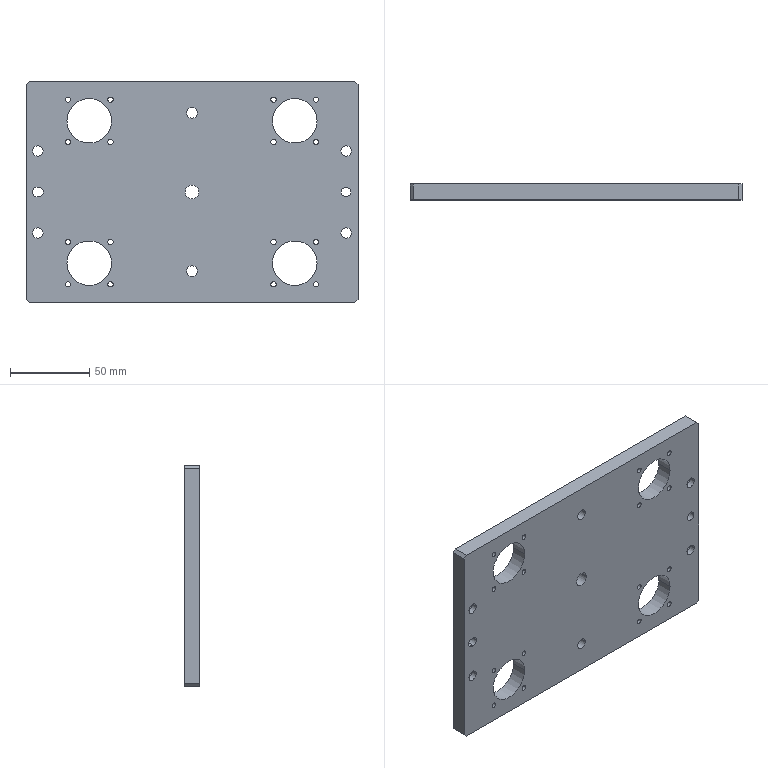Component | SolidWorks | 20-MaterialTrayLifting-1111-1_21-1111-1 | 1 solid | 83 faces | box 210 x 10 x 140 mm | volume 262683 mm3 | cylinder 67 | plane 16 | commonest cylinder face diameters 3.3 x32 11 x8 6.6 x8 28.2 x8 6 x5 6.8 x4 8.8 x2 | material S45C
build123d program:
from build123d import *

# Parameters (mm, degrees)
SKETCH1_W                                       = 210
SKETCH1_H                                       = 140
BOSS_EXTRUDE1_DEPTH                             = 10
SKETCH2_R                                       = 14.1
CUT_EXTRUDE1_DEPTH                              = 127.59
SKETCH5_R                                       = 3
CUT_EXTRUDE2_DEPTH                              = 127.59
M6_HEX_SOCKET_HEAD_CAP_SCREW_CBORE1_D           = 6.6
M6_HEX_SOCKET_HEAD_CAP_SCREW_CBORE1_CBORE_D     = 11
M6_HEX_SOCKET_HEAD_CAP_SCREW_CBORE1_CBORE_DEPTH = 6.4
SIZE_MM_DOWEL_PIN_HOLE_1_D                      = 6
CHAMFER1_SIZE                                   = 2
CUT_EXTRUDE4_DEPTH                              = 127.59
M8_TAPPED_HOLE1_D                               = 6.8
M4_TAPPED_HOLE1_AT_2_COUNT                      = 2
M4_TAPPED_HOLE1_AT_2_PITCH                      = 26.87
M4_TAPPED_HOLE1_AT_3_COUNT                      = 2
M4_TAPPED_HOLE1_AT_3_PITCH                      = 38
M4_TAPPED_HOLE1_AT_4_COUNT                      = 2
M4_TAPPED_HOLE1_AT_4_PITCH                      = 26.87
M10X1_25_TAPPED_HOLE1_D                         = 8.8


with BuildPart() as part:
    # Sketch1 → Boss-Extrude1 (new body)
    with BuildSketch(Plane.XY):
        Rectangle(SKETCH1_W, SKETCH1_H)
    extrude(amount=BOSS_EXTRUDE1_DEPTH)

    # Sketch2 → Cut-Extrude1 (cut, through all)
    with BuildSketch(Plane.XY.offset(10)):
        with Locations((-65, 45)):
            Circle(SKETCH2_R)
        with Locations((65, 45)):
            Circle(SKETCH2_R)
        with Locations((-65, -45)):
            Circle(SKETCH2_R)
        with Locations((65, -45)):
            Circle(SKETCH2_R)
    extrude(amount=-CUT_EXTRUDE1_DEPTH, mode=Mode.SUBTRACT)

    # Sketch5 → Cut-Extrude2 (cut, through all)
    with BuildSketch(Plane.XY.offset(10)):
        Circle(SKETCH5_R)
    extrude(amount=-CUT_EXTRUDE2_DEPTH, mode=Mode.SUBTRACT)

    # M6 Hex Socket Head Cap Screw CBORE1 (through all)
    with Locations(Plane.XY.offset(10)):
        with Locations((-97.5, 78), (-97.5, 26), (-97.5, -26), (-97.5, -78), (97.5, 78), (97.5, 26), (97.5, -26), (97.5, -78)):
            CounterBoreHole(M6_HEX_SOCKET_HEAD_CAP_SCREW_CBORE1_D / 2, M6_HEX_SOCKET_HEAD_CAP_SCREW_CBORE1_CBORE_D / 2, M6_HEX_SOCKET_HEAD_CAP_SCREW_CBORE1_CBORE_DEPTH)

    # Size mm Dowel Pin Hole 1 (through all)
    with Locations(Plane.XY.offset(10)):
        with Locations((-97.5, 0), (97.5, 0)):
            Hole(SIZE_MM_DOWEL_PIN_HOLE_1_D / 2)

    # Chamfer1
    chamfer1_edges = [part.edges().sort_by_distance(p)[0] for p in [
        (105, -70, 5),
        (-105, -70, 5),
        (-105, 70, 5),
        (105, 70, 5),
    ]]
    chamfer(chamfer1_edges, length=CHAMFER1_SIZE)

    # Sketch17 → Cut-Extrude4 (cut, through all)
    with BuildSketch(Plane.XY.offset(10)):
        with BuildLine():
            Line((-98, 3), (-97, 3))
            ThreePointArc((-97, 3), (-94, 0), (-97, -3))
            Line((-97, -3), (-98, -3))
            ThreePointArc((-98, -3), (-101, 0), (-98, 3))
        make_face()
    extrude(amount=-CUT_EXTRUDE4_DEPTH, mode=Mode.SUBTRACT)

    # M8 Tapped Hole1 (through all)
    with Locations(Plane.XY.offset(10)):
        with Locations((0, -50), (0, 50)):
            Hole(M8_TAPPED_HOLE1_D / 2)

    # Sketch23 → M4 Tapped Hole1 (revolve, cut)
    with BuildSketch(Plane(origin=(-78.435, -31.565, 10), x_dir=(0, -1, 0), z_dir=(1, 0, 0))):
        Polygon((0, 0), (0, 11.091), (1.65, 10.1), (1.65, 0), align=None)
    m4_tapped_hole1 = revolve(axis=Axis((-78.435, -31.565, 16.35), (0, 0, -1)), mode=Mode.SUBTRACT)

    # M4 Tapped Hole1 at 2: M4 Tapped Hole1 ×2
    with Locations(*[(0, -i * M4_TAPPED_HOLE1_AT_2_PITCH, 0) for i in range(1, M4_TAPPED_HOLE1_AT_2_COUNT)]):
        add(m4_tapped_hole1, mode=Mode.SUBTRACT)

    # M4 Tapped Hole1 at 3: M4 Tapped Hole1 ×2
    with Locations(*[Vector(0.7071, -0.7071, 0) * (i * M4_TAPPED_HOLE1_AT_3_PITCH) for i in range(1, M4_TAPPED_HOLE1_AT_3_COUNT)]):
        add(m4_tapped_hole1, mode=Mode.SUBTRACT)

    # M4 Tapped Hole1 at 4: M4 Tapped Hole1 ×2
    with Locations(*[(i * M4_TAPPED_HOLE1_AT_4_PITCH, 0, 0) for i in range(1, M4_TAPPED_HOLE1_AT_4_COUNT)]):
        add(m4_tapped_hole1, mode=Mode.SUBTRACT)

    # Mirror1: M4 Tapped Hole1 across plane
    add(m4_tapped_hole1.mirror(Plane.ZX), mode=Mode.SUBTRACT)

    # Mirror1 copy 1 sketch → Mirror1 copy 1 (revolve, cut)
    with BuildSketch(Plane(origin=(-78.435, 58.435, 10), x_dir=(0, 1, 0), z_dir=(1, 0, 0))):
        Polygon((0, 0), (0, -11.091), (1.65, -10.1), (1.65, 0), align=None)
    revolve(axis=Axis((-78.435, 58.435, 16.35), (0, 0, 1)), mode=Mode.SUBTRACT)

    # Mirror1 copy 2 sketch → Mirror1 copy 2 (revolve, cut)
    with BuildSketch(Plane(origin=(-51.565, 58.435, 10), x_dir=(0, 1, 0), z_dir=(1, 0, 0))):
        Polygon((0, 0), (0, -11.091), (1.65, -10.1), (1.65, 0), align=None)
    revolve(axis=Axis((-51.565, 58.435, 16.35), (0, 0, 1)), mode=Mode.SUBTRACT)

    # Mirror1 copy 3 sketch → Mirror1 copy 3 (revolve, cut)
    with BuildSketch(Plane(origin=(-51.565, 31.565, 10), x_dir=(0, 1, 0), z_dir=(1, 0, 0))):
        Polygon((0, 0), (0, -11.091), (1.65, -10.1), (1.65, 0), align=None)
    revolve(axis=Axis((-51.565, 31.565, 16.35), (0, 0, 1)), mode=Mode.SUBTRACT)

    # Mirror2: M4 Tapped Hole1 across plane
    add(m4_tapped_hole1.mirror(Plane(origin=(0, 0, 0), x_dir=(0, 0, 1), z_dir=(1, 0, 0))), mode=Mode.SUBTRACT)

    # Mirror2 copy 1 sketch → Mirror2 copy 1 (revolve, cut)
    with BuildSketch(Plane(origin=(78.435, -58.435, 10), x_dir=(0, -1, 0), z_dir=(-1, 0, 0))):
        Polygon((0, 0), (0, -11.091), (1.65, -10.1), (1.65, 0), align=None)
    revolve(axis=Axis((78.435, -58.435, 16.35), (0, 0, 1)), mode=Mode.SUBTRACT)

    # Mirror2 copy 2 sketch → Mirror2 copy 2 (revolve, cut)
    with BuildSketch(Plane(origin=(51.565, -58.435, 10), x_dir=(0, -1, 0), z_dir=(-1, 0, 0))):
        Polygon((0, 0), (0, -11.091), (1.65, -10.1), (1.65, 0), align=None)
    revolve(axis=Axis((51.565, -58.435, 16.35), (0, 0, 1)), mode=Mode.SUBTRACT)

    # Mirror2 copy 3 sketch → Mirror2 copy 3 (revolve, cut)
    with BuildSketch(Plane(origin=(51.565, -31.565, 10), x_dir=(0, -1, 0), z_dir=(-1, 0, 0))):
        Polygon((0, 0), (0, -11.091), (1.65, -10.1), (1.65, 0), align=None)
    revolve(axis=Axis((51.565, -31.565, 16.35), (0, 0, 1)), mode=Mode.SUBTRACT)

    # Mirror2 copy 4 sketch → Mirror2 copy 4 (revolve, cut)
    with BuildSketch(Plane(origin=(78.435, 31.565, 10), x_dir=(0, 1, 0), z_dir=(-1, 0, 0))):
        Polygon((0, 0), (0, 11.091), (1.65, 10.1), (1.65, 0), align=None)
    revolve(axis=Axis((78.435, 31.565, 16.35), (0, 0, -1)), mode=Mode.SUBTRACT)

    # Mirror2 copy 5 sketch → Mirror2 copy 5 (revolve, cut)
    with BuildSketch(Plane(origin=(78.435, 58.435, 10), x_dir=(0, 1, 0), z_dir=(-1, 0, 0))):
        Polygon((0, 0), (0, 11.091), (1.65, 10.1), (1.65, 0), align=None)
    revolve(axis=Axis((78.435, 58.435, 16.35), (0, 0, -1)), mode=Mode.SUBTRACT)

    # Mirror2 copy 6 sketch → Mirror2 copy 6 (revolve, cut)
    with BuildSketch(Plane(origin=(51.565, 58.435, 10), x_dir=(0, 1, 0), z_dir=(-1, 0, 0))):
        Polygon((0, 0), (0, 11.091), (1.65, 10.1), (1.65, 0), align=None)
    revolve(axis=Axis((51.565, 58.435, 16.35), (0, 0, -1)), mode=Mode.SUBTRACT)

    # Mirror2 copy 7 sketch → Mirror2 copy 7 (revolve, cut)
    with BuildSketch(Plane(origin=(51.565, 31.565, 10), x_dir=(0, 1, 0), z_dir=(-1, 0, 0))):
        Polygon((0, 0), (0, 11.091), (1.65, 10.1), (1.65, 0), align=None)
    revolve(axis=Axis((51.565, 31.565, 16.35), (0, 0, -1)), mode=Mode.SUBTRACT)

    # M10x1.25 Tapped Hole1 (through all)
    with Locations(Plane.XY.offset(10)):
        with Locations((0, 0)):
            Hole(M10X1_25_TAPPED_HOLE1_D / 2)


solid = part.part

# Placed as in the assembly
solid = solid.moved(Location((3.428, 396.224, 1393.056), (-90, 0, 0)))